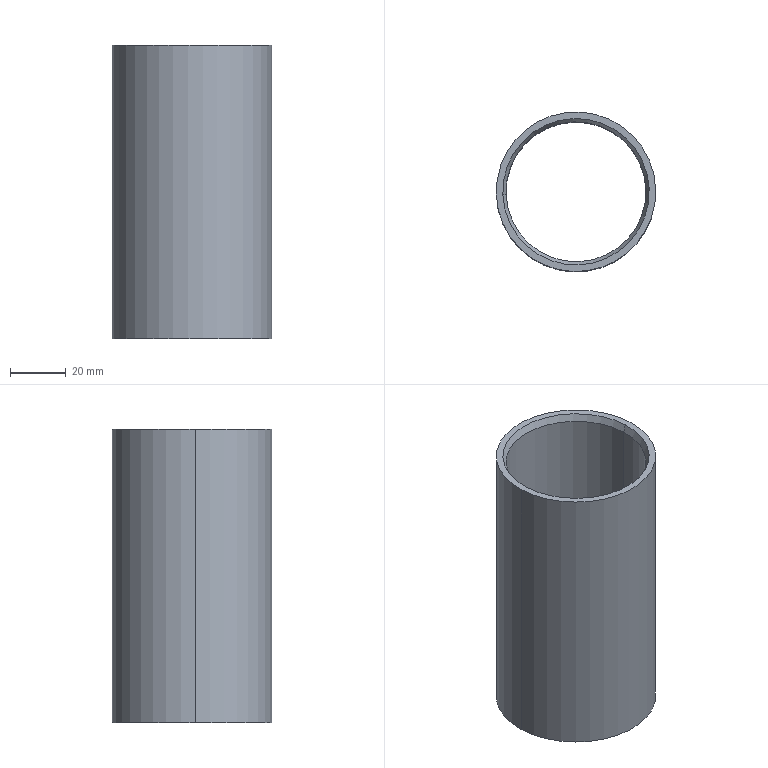Component | SolidWorks | Cylinder-1_SteelBarrel-1 | 1 solid | 10 faces | box 57 x 57 x 105 mm | volume 61303 mm3 | cone 4 | cylinder 4 | plane 2 | commonest cylinder face diameters 50 x2 57 x2
build123d program:
from build123d import *

# Parameters (mm, degrees)
SKETCH1_R           = 28.5
SKETCH1_R_2         = 25
BOSS_EXTRUDE1_DEPTH = 105
CHAMFER1_SIZE       = 2.5
CHAMFER1_SIZE2      = 1.166


with BuildPart() as part:
    # Sketch1 → Boss-Extrude1 (new body)
    with BuildSketch(Plane.XY):
        Circle(SKETCH1_R)
        Circle(SKETCH1_R_2, mode=Mode.SUBTRACT)
    extrude(amount=BOSS_EXTRUDE1_DEPTH)

    # Chamfer1
    chamfer1_edges = [part.edges().sort_by_distance(p)[0] for p in [
        (-25, 0, 0),
        (-25, 0, 105),
    ]]
    chamfer1_side = [part.faces().sort_by_distance(p)[0] for p in [
        (-25, 0, 52.5),
    ]]
    chamfer(chamfer1_edges, length=CHAMFER1_SIZE, length2=CHAMFER1_SIZE2, reference=chamfer1_side[0])


solid = part.part

# Placed as in the assembly
solid = solid.moved(Location((-180.557, 26.412, -337.351), (0, 0, 0)))
STEP:
#1=COLOUR_RGB('',0.7922,0.8196,0.9333);
#2=FILL_AREA_STYLE_COLOUR('',#1);
#3=FILL_AREA_STYLE('',(#2));
#4=SURFACE_STYLE_FILL_AREA(#3);
#5=SURFACE_SIDE_STYLE('',(#4));
#6=SURFACE_STYLE_USAGE(.BOTH.,#5);
#7=PRESENTATION_STYLE_ASSIGNMENT((#6));
#8=CARTESIAN_POINT('',(-6.125,1.08,-9.246));
#9=VERTEX_POINT('',#8);
#10=CARTESIAN_POINT('',(-8.092,0.9995,-9.246));
#11=VERTEX_POINT('',#10);
#12=CARTESIAN_POINT('',(-7.109,1.04,-9.246));
#13=DIRECTION('',(-0.,0.,1.));
#14=DIRECTION('',(-0.9992,-0.04098,0.));
#15=AXIS2_PLACEMENT_3D('',#12,#13,#14);
#16=CIRCLE('',#15,0.9843);
#17=EDGE_CURVE('',#9,#11,#16,.T.);
#18=ORIENTED_EDGE('',*,*,#17,.F.);
#19=CARTESIAN_POINT('',(-6.079,1.082,-9.148));
#20=VERTEX_POINT('',#19);
#21=CARTESIAN_POINT('',(-6.125,1.08,-9.246));
#22=DIRECTION('',(0.4223,0.01732,0.9063));
#23=VECTOR('',#22,39.37);
#24=LINE('',#21,#23);
#25=EDGE_CURVE('',#9,#20,#24,.T.);
#26=ORIENTED_EDGE('',*,*,#25,.T.);
#27=CARTESIAN_POINT('',(-8.138,0.9976,-9.148));
#28=VERTEX_POINT('',#27);
#29=CARTESIAN_POINT('',(-7.109,1.04,-9.148));
#30=DIRECTION('',(0.,-0.,-1.));
#31=DIRECTION('',(-0.9992,-0.04098,0.));
#32=AXIS2_PLACEMENT_3D('',#29,#30,#31);
#33=CIRCLE('',#32,1.03);
#34=EDGE_CURVE('',#28,#20,#33,.T.);
#35=ORIENTED_EDGE('',*,*,#34,.F.);
#36=CARTESIAN_POINT('',(-8.092,0.9995,-9.246));
#37=DIRECTION('',(-0.4223,-0.01732,0.9063));
#38=VECTOR('',#37,39.37);
#39=LINE('',#36,#38);
#40=EDGE_CURVE('',#11,#28,#39,.T.);
#41=ORIENTED_EDGE('',*,*,#40,.F.);
#42=EDGE_LOOP('',(#18,#26,#35,#41));
#43=FACE_OUTER_BOUND('',#42,.T.);
#44=CARTESIAN_POINT('',(-7.109,1.04,-9.246));
#45=DIRECTION('',(-0.,0.,1.));
#46=DIRECTION('',(-0.9992,-0.04098,0.));
#47=AXIS2_PLACEMENT_3D('',#44,#45,#46);
#48=CONICAL_SURFACE('',#47,0.9843,0.4363);
#49=ADVANCED_FACE('',(#43),#48,.F.);
#50=CARTESIAN_POINT('',(-8.092,0.9995,-13.183));
#51=VERTEX_POINT('',#50);
#52=CARTESIAN_POINT('',(-6.125,1.08,-13.183));
#53=VERTEX_POINT('',#52);
#54=CARTESIAN_POINT('',(-7.109,1.04,-13.183));
#55=DIRECTION('',(0.,-0.,-1.));
#56=DIRECTION('',(-0.9992,-0.04098,0.));
#57=AXIS2_PLACEMENT_3D('',#54,#55,#56);
#58=CIRCLE('',#57,0.9843);
#59=EDGE_CURVE('',#51,#53,#58,.T.);
#60=ORIENTED_EDGE('',*,*,#59,.F.);
#61=CARTESIAN_POINT('',(-8.138,0.9976,-13.282));
#62=VERTEX_POINT('',#61);
#63=CARTESIAN_POINT('',(-8.138,0.9976,-13.282));
#64=DIRECTION('',(-0.4223,-0.01732,-0.9063));
#65=VECTOR('',#64,39.37);
#66=LINE('',#63,#65);
#67=EDGE_CURVE('',#51,#62,#66,.T.);
#68=ORIENTED_EDGE('',*,*,#67,.T.);
#69=CARTESIAN_POINT('',(-6.079,1.082,-13.282));
#70=VERTEX_POINT('',#69);
#71=CARTESIAN_POINT('',(-7.109,1.04,-13.282));
#72=DIRECTION('',(-0.,0.,1.));
#73=DIRECTION('',(-0.9992,-0.04098,0.));
#74=AXIS2_PLACEMENT_3D('',#71,#72,#73);
#75=CIRCLE('',#74,1.03);
#76=EDGE_CURVE('',#70,#62,#75,.T.);
#77=ORIENTED_EDGE('',*,*,#76,.F.);
#78=CARTESIAN_POINT('',(-6.079,1.082,-13.282));
#79=DIRECTION('',(0.4223,0.01732,-0.9063));
#80=VECTOR('',#79,39.37);
#81=LINE('',#78,#80);
#82=EDGE_CURVE('',#53,#70,#81,.T.);
#83=ORIENTED_EDGE('',*,*,#82,.F.);
#84=EDGE_LOOP('',(#60,#68,#77,#83));
#85=FACE_OUTER_BOUND('',#84,.T.);
#86=CARTESIAN_POINT('',(-7.109,1.04,-13.282));
#87=DIRECTION('',(0.,-0.,-1.));
#88=DIRECTION('',(0.9992,0.04098,0.));
#89=AXIS2_PLACEMENT_3D('',#86,#87,#88);
#90=CONICAL_SURFACE('',#89,1.03,0.4363);
#91=ADVANCED_FACE('',(#85),#90,.F.);
#92=ORIENTED_EDGE('',*,*,#17,.T.);
#93=CARTESIAN_POINT('',(-8.092,0.9995,-9.148));
#94=DIRECTION('',(0.,-0.,-1.));
#95=VECTOR('',#94,39.37);
#96=LINE('',#93,#95);
#97=EDGE_CURVE('',#11,#51,#96,.T.);
#98=ORIENTED_EDGE('',*,*,#97,.T.);
#99=ORIENTED_EDGE('',*,*,#59,.T.);
#100=CARTESIAN_POINT('',(-6.125,1.08,-9.148));
#101=DIRECTION('',(0.,-0.,-1.));
#102=VECTOR('',#101,39.37);
#103=LINE('',#100,#102);
#104=EDGE_CURVE('',#9,#53,#103,.T.);
#105=ORIENTED_EDGE('',*,*,#104,.F.);
#106=EDGE_LOOP('',(#92,#98,#99,#105));
#107=FACE_OUTER_BOUND('',#106,.T.);
#108=CARTESIAN_POINT('',(-7.109,1.04,-9.148));
#109=DIRECTION('',(0.,-0.,-1.));
#110=DIRECTION('',(0.9992,0.04098,0.));
#111=AXIS2_PLACEMENT_3D('',#108,#109,#110);
#112=CYLINDRICAL_SURFACE('',#111,0.9843);
#113=ADVANCED_FACE('',(#107),#112,.F.);
#114=CARTESIAN_POINT('',(-8.23,0.9939,-9.148));
#115=VERTEX_POINT('',#114);
#116=CARTESIAN_POINT('',(-5.987,1.086,-9.148));
#117=VERTEX_POINT('',#116);
#118=CARTESIAN_POINT('',(-7.109,1.04,-9.148));
#119=DIRECTION('',(-0.,0.,1.));
#120=DIRECTION('',(-0.9992,-0.04098,0.));
#121=AXIS2_PLACEMENT_3D('',#118,#119,#120);
#122=CIRCLE('',#121,1.122);
#123=EDGE_CURVE('',#115,#117,#122,.T.);
#124=ORIENTED_EDGE('',*,*,#123,.F.);
#125=CARTESIAN_POINT('',(-8.23,0.9939,-13.282));
#126=VERTEX_POINT('',#125);
#127=CARTESIAN_POINT('',(-8.23,0.9939,-9.148));
#128=DIRECTION('',(0.,-0.,-1.));
#129=VECTOR('',#128,39.37);
#130=LINE('',#127,#129);
#131=EDGE_CURVE('',#115,#126,#130,.T.);
#132=ORIENTED_EDGE('',*,*,#131,.T.);
#133=CARTESIAN_POINT('',(-5.987,1.086,-13.282));
#134=VERTEX_POINT('',#133);
#135=CARTESIAN_POINT('',(-7.109,1.04,-13.282));
#136=DIRECTION('',(-0.,0.,1.));
#137=DIRECTION('',(-0.9992,-0.04098,0.));
#138=AXIS2_PLACEMENT_3D('',#135,#136,#137);
#139=CIRCLE('',#138,1.122);
#140=EDGE_CURVE('',#126,#134,#139,.T.);
#141=ORIENTED_EDGE('',*,*,#140,.T.);
#142=CARTESIAN_POINT('',(-5.987,1.086,-9.148));
#143=DIRECTION('',(0.,-0.,-1.));
#144=VECTOR('',#143,39.37);
#145=LINE('',#142,#144);
#146=EDGE_CURVE('',#117,#134,#145,.T.);
#147=ORIENTED_EDGE('',*,*,#146,.F.);
#148=EDGE_LOOP('',(#124,#132,#141,#147));
#149=FACE_OUTER_BOUND('',#148,.T.);
#150=CARTESIAN_POINT('',(-7.109,1.04,-9.148));
#151=DIRECTION('',(0.,-0.,-1.));
#152=DIRECTION('',(0.9992,0.04098,0.));
#153=AXIS2_PLACEMENT_3D('',#150,#151,#152);
#154=CYLINDRICAL_SURFACE('',#153,1.122);
#155=ADVANCED_FACE('',(#149),#154,.T.);
#156=ORIENTED_EDGE('',*,*,#34,.T.);
#157=CARTESIAN_POINT('',(-7.109,1.04,-9.148));
#158=DIRECTION('',(0.,-0.,-1.));
#159=DIRECTION('',(-0.9992,-0.04098,0.));
#160=AXIS2_PLACEMENT_3D('',#157,#158,#159);
#161=CIRCLE('',#160,1.03);
#162=EDGE_CURVE('',#20,#28,#161,.T.);
#163=ORIENTED_EDGE('',*,*,#162,.T.);
#164=EDGE_LOOP('',(#156,#163));
#165=FACE_BOUND('',#164,.T.);
#166=CARTESIAN_POINT('',(-7.109,1.04,-9.148));
#167=DIRECTION('',(-0.,0.,1.));
#168=DIRECTION('',(-0.9992,-0.04098,0.));
#169=AXIS2_PLACEMENT_3D('',#166,#167,#168);
#170=CIRCLE('',#169,1.122);
#171=EDGE_CURVE('',#117,#115,#170,.T.);
#172=ORIENTED_EDGE('',*,*,#171,.T.);
#173=ORIENTED_EDGE('',*,*,#123,.T.);
#174=EDGE_LOOP('',(#172,#173));
#175=FACE_OUTER_BOUND('',#174,.T.);
#176=CARTESIAN_POINT('',(-7.109,1.04,-9.148));
#177=DIRECTION('',(-0.,0.,1.));
#178=DIRECTION('',(-0.9992,-0.04098,0.));
#179=AXIS2_PLACEMENT_3D('',#176,#177,#178);
#180=PLANE('',#179);
#181=ADVANCED_FACE('',(#165,#175),#180,.T.);
#182=ORIENTED_EDGE('',*,*,#76,.T.);
#183=CARTESIAN_POINT('',(-7.109,1.04,-13.282));
#184=DIRECTION('',(-0.,0.,1.));
#185=DIRECTION('',(-0.9992,-0.04098,0.));
#186=AXIS2_PLACEMENT_3D('',#183,#184,#185);
#187=CIRCLE('',#186,1.03);
#188=EDGE_CURVE('',#62,#70,#187,.T.);
#189=ORIENTED_EDGE('',*,*,#188,.T.);
#190=EDGE_LOOP('',(#182,#189));
#191=FACE_BOUND('',#190,.T.);
#192=CARTESIAN_POINT('',(-7.109,1.04,-13.282));
#193=DIRECTION('',(-0.,0.,1.));
#194=DIRECTION('',(-0.9992,-0.04098,0.));
#195=AXIS2_PLACEMENT_3D('',#192,#193,#194);
#196=CIRCLE('',#195,1.122);
#197=EDGE_CURVE('',#134,#126,#196,.T.);
#198=ORIENTED_EDGE('',*,*,#197,.F.);
#199=ORIENTED_EDGE('',*,*,#140,.F.);
#200=EDGE_LOOP('',(#198,#199));
#201=FACE_OUTER_BOUND('',#200,.T.);
#202=CARTESIAN_POINT('',(-7.109,1.04,-13.282));
#203=DIRECTION('',(-0.,0.,1.));
#204=DIRECTION('',(-0.9992,-0.04098,0.));
#205=AXIS2_PLACEMENT_3D('',#202,#203,#204);
#206=PLANE('',#205);
#207=ADVANCED_FACE('',(#191,#201),#206,.F.);
#208=ORIENTED_EDGE('',*,*,#131,.F.);
#209=ORIENTED_EDGE('',*,*,#171,.F.);
#210=ORIENTED_EDGE('',*,*,#146,.T.);
#211=ORIENTED_EDGE('',*,*,#197,.T.);
#212=EDGE_LOOP('',(#208,#209,#210,#211));
#213=FACE_OUTER_BOUND('',#212,.T.);
#214=CARTESIAN_POINT('',(-7.109,1.04,-9.148));
#215=DIRECTION('',(0.,-0.,-1.));
#216=DIRECTION('',(0.9992,0.04098,0.));
#217=AXIS2_PLACEMENT_3D('',#214,#215,#216);
#218=CYLINDRICAL_SURFACE('',#217,1.122);
#219=ADVANCED_FACE('',(#213),#218,.T.);
#220=ORIENTED_EDGE('',*,*,#97,.F.);
#221=CARTESIAN_POINT('',(-7.109,1.04,-9.246));
#222=DIRECTION('',(-0.,0.,1.));
#223=DIRECTION('',(-0.9992,-0.04098,0.));
#224=AXIS2_PLACEMENT_3D('',#221,#222,#223);
#225=CIRCLE('',#224,0.9843);
#226=EDGE_CURVE('',#11,#9,#225,.T.);
#227=ORIENTED_EDGE('',*,*,#226,.T.);
#228=ORIENTED_EDGE('',*,*,#104,.T.);
#229=CARTESIAN_POINT('',(-7.109,1.04,-13.183));
#230=DIRECTION('',(0.,-0.,-1.));
#231=DIRECTION('',(-0.9992,-0.04098,0.));
#232=AXIS2_PLACEMENT_3D('',#229,#230,#231);
#233=CIRCLE('',#232,0.9843);
#234=EDGE_CURVE('',#53,#51,#233,.T.);
#235=ORIENTED_EDGE('',*,*,#234,.T.);
#236=EDGE_LOOP('',(#220,#227,#228,#235));
#237=FACE_OUTER_BOUND('',#236,.T.);
#238=CARTESIAN_POINT('',(-7.109,1.04,-9.148));
#239=DIRECTION('',(0.,-0.,-1.));
#240=DIRECTION('',(0.9992,0.04098,0.));
#241=AXIS2_PLACEMENT_3D('',#238,#239,#240);
#242=CYLINDRICAL_SURFACE('',#241,0.9843);
#243=ADVANCED_FACE('',(#237),#242,.F.);
#244=ORIENTED_EDGE('',*,*,#67,.F.);
#245=ORIENTED_EDGE('',*,*,#234,.F.);
#246=ORIENTED_EDGE('',*,*,#82,.T.);
#247=ORIENTED_EDGE('',*,*,#188,.F.);
#248=EDGE_LOOP('',(#244,#245,#246,#247));
#249=FACE_OUTER_BOUND('',#248,.T.);
#250=CARTESIAN_POINT('',(-7.109,1.04,-13.282));
#251=DIRECTION('',(0.,-0.,-1.));
#252=DIRECTION('',(0.9992,0.04098,0.));
#253=AXIS2_PLACEMENT_3D('',#250,#251,#252);
#254=CONICAL_SURFACE('',#253,1.03,0.4363);
#255=ADVANCED_FACE('',(#249),#254,.F.);
#256=ORIENTED_EDGE('',*,*,#25,.F.);
#257=ORIENTED_EDGE('',*,*,#226,.F.);
#258=ORIENTED_EDGE('',*,*,#40,.T.);
#259=ORIENTED_EDGE('',*,*,#162,.F.);
#260=EDGE_LOOP('',(#256,#257,#258,#259));
#261=FACE_OUTER_BOUND('',#260,.T.);
#262=CARTESIAN_POINT('',(-7.109,1.04,-9.246));
#263=DIRECTION('',(-0.,0.,1.));
#264=DIRECTION('',(-0.9992,-0.04098,0.));
#265=AXIS2_PLACEMENT_3D('',#262,#263,#264);
#266=CONICAL_SURFACE('',#265,0.9843,0.4363);
#267=ADVANCED_FACE('',(#261),#266,.F.);
#268=CLOSED_SHELL('',(#49,#91,#113,#155,#181,#207,#219,#243,#255,#267));
#269=MANIFOLD_SOLID_BREP('',#268);
#270=STYLED_ITEM('',(#7),#269);
#271=(LENGTH_UNIT()NAMED_UNIT(*)SI_UNIT($,.METRE.));
#272=LENGTH_MEASURE_WITH_UNIT(LENGTH_MEASURE(0.0254),#271);
#273=DIMENSIONAL_EXPONENTS(1.,0.,0.,0.,0.,0.,0.);
#274=(CONVERSION_BASED_UNIT('',#272)LENGTH_UNIT()NAMED_UNIT(#273));
#275=UNCERTAINTY_MEASURE_WITH_UNIT(LENGTH_MEASURE(0.00001),#274,'','');
#276=(NAMED_UNIT(*)PLANE_ANGLE_UNIT()SI_UNIT($,.RADIAN.));
#277=(NAMED_UNIT(*)SI_UNIT($,.STERADIAN.)SOLID_ANGLE_UNIT());
#278=(GEOMETRIC_REPRESENTATION_CONTEXT(3)GLOBAL_UNCERTAINTY_ASSIGNED_CONTEXT((#275))GLOBAL_UNIT_ASSIGNED_CONTEXT((#274,#276,#277))REPRESENTATION_CONTEXT('',''));
#279=MECHANICAL_DESIGN_GEOMETRIC_PRESENTATION_REPRESENTATION('',(#270),#278);
#280=PRESENTATION_LAYER_ASSIGNMENT('','',(#270));
#281=CARTESIAN_POINT('',(0.,0.,0.));
#282=DIRECTION('',(0.,0.,1.));
#283=DIRECTION('',(1.,0.,0.));
#284=AXIS2_PLACEMENT_3D('',#281,#282,#283);
#285=(LENGTH_UNIT()NAMED_UNIT(*)SI_UNIT($,.METRE.));
#286=LENGTH_MEASURE_WITH_UNIT(LENGTH_MEASURE(0.0254),#285);
#287=DIMENSIONAL_EXPONENTS(1.,0.,0.,0.,0.,0.,0.);
#288=(CONVERSION_BASED_UNIT('',#286)LENGTH_UNIT()NAMED_UNIT(#287));
#289=UNCERTAINTY_MEASURE_WITH_UNIT(LENGTH_MEASURE(0.00001),#288,'','');
#290=(NAMED_UNIT(*)PLANE_ANGLE_UNIT()SI_UNIT($,.RADIAN.));
#291=(NAMED_UNIT(*)SI_UNIT($,.STERADIAN.)SOLID_ANGLE_UNIT());
#292=(GEOMETRIC_REPRESENTATION_CONTEXT(3)GLOBAL_UNCERTAINTY_ASSIGNED_CONTEXT((#289))GLOBAL_UNIT_ASSIGNED_CONTEXT((#288,#290,#291))REPRESENTATION_CONTEXT('',''));
#293=ADVANCED_BREP_SHAPE_REPRESENTATION('',(#269,#284),#292);